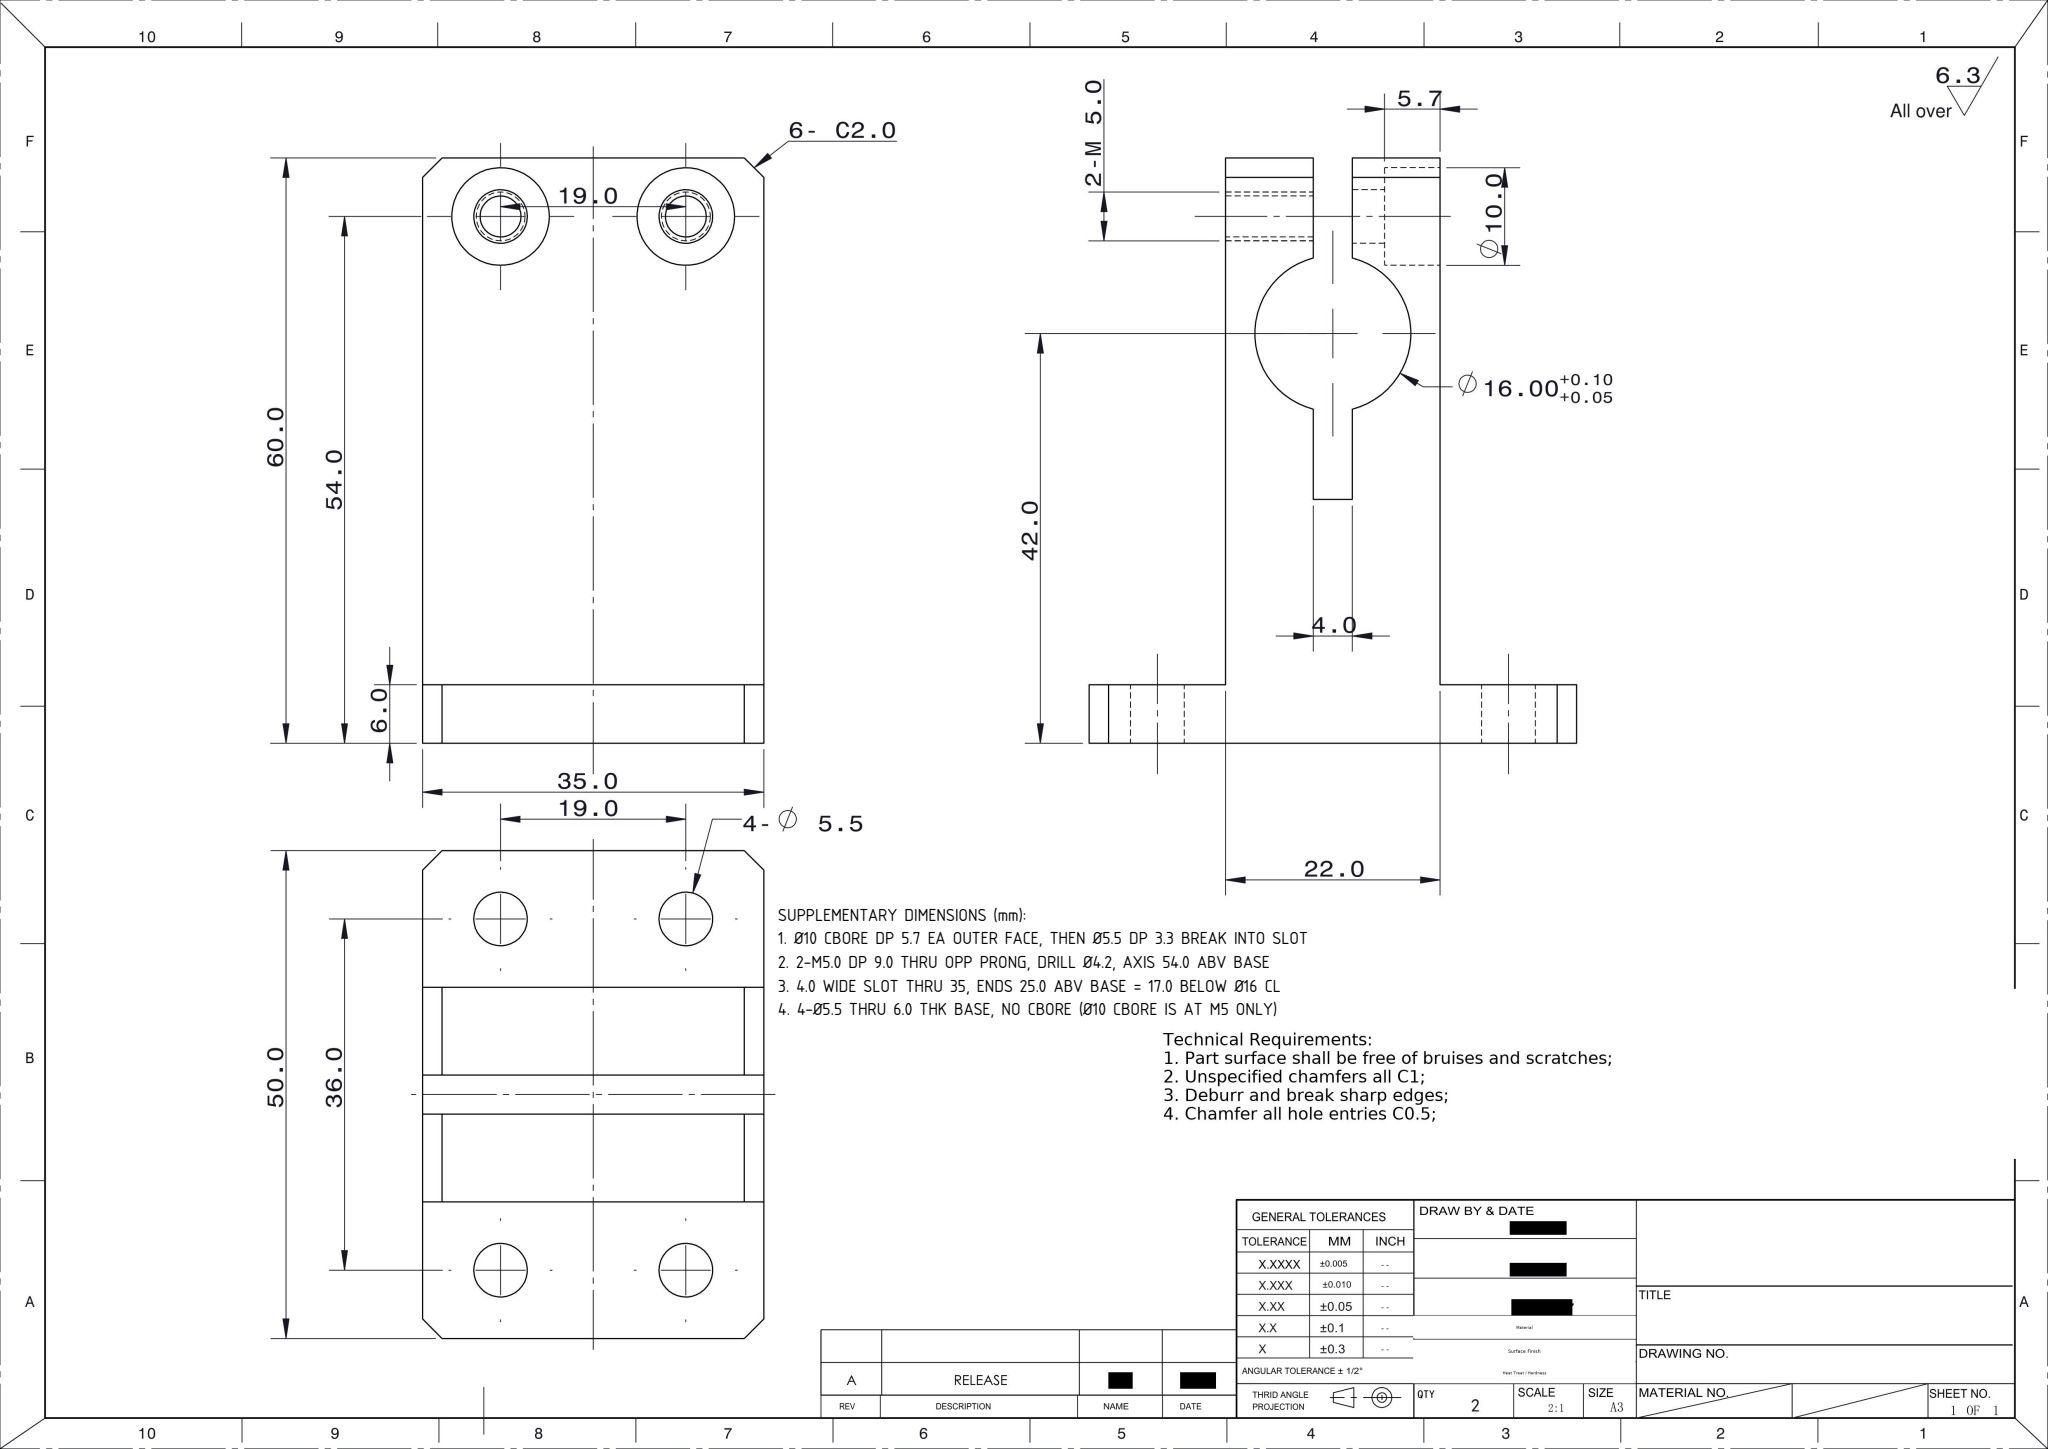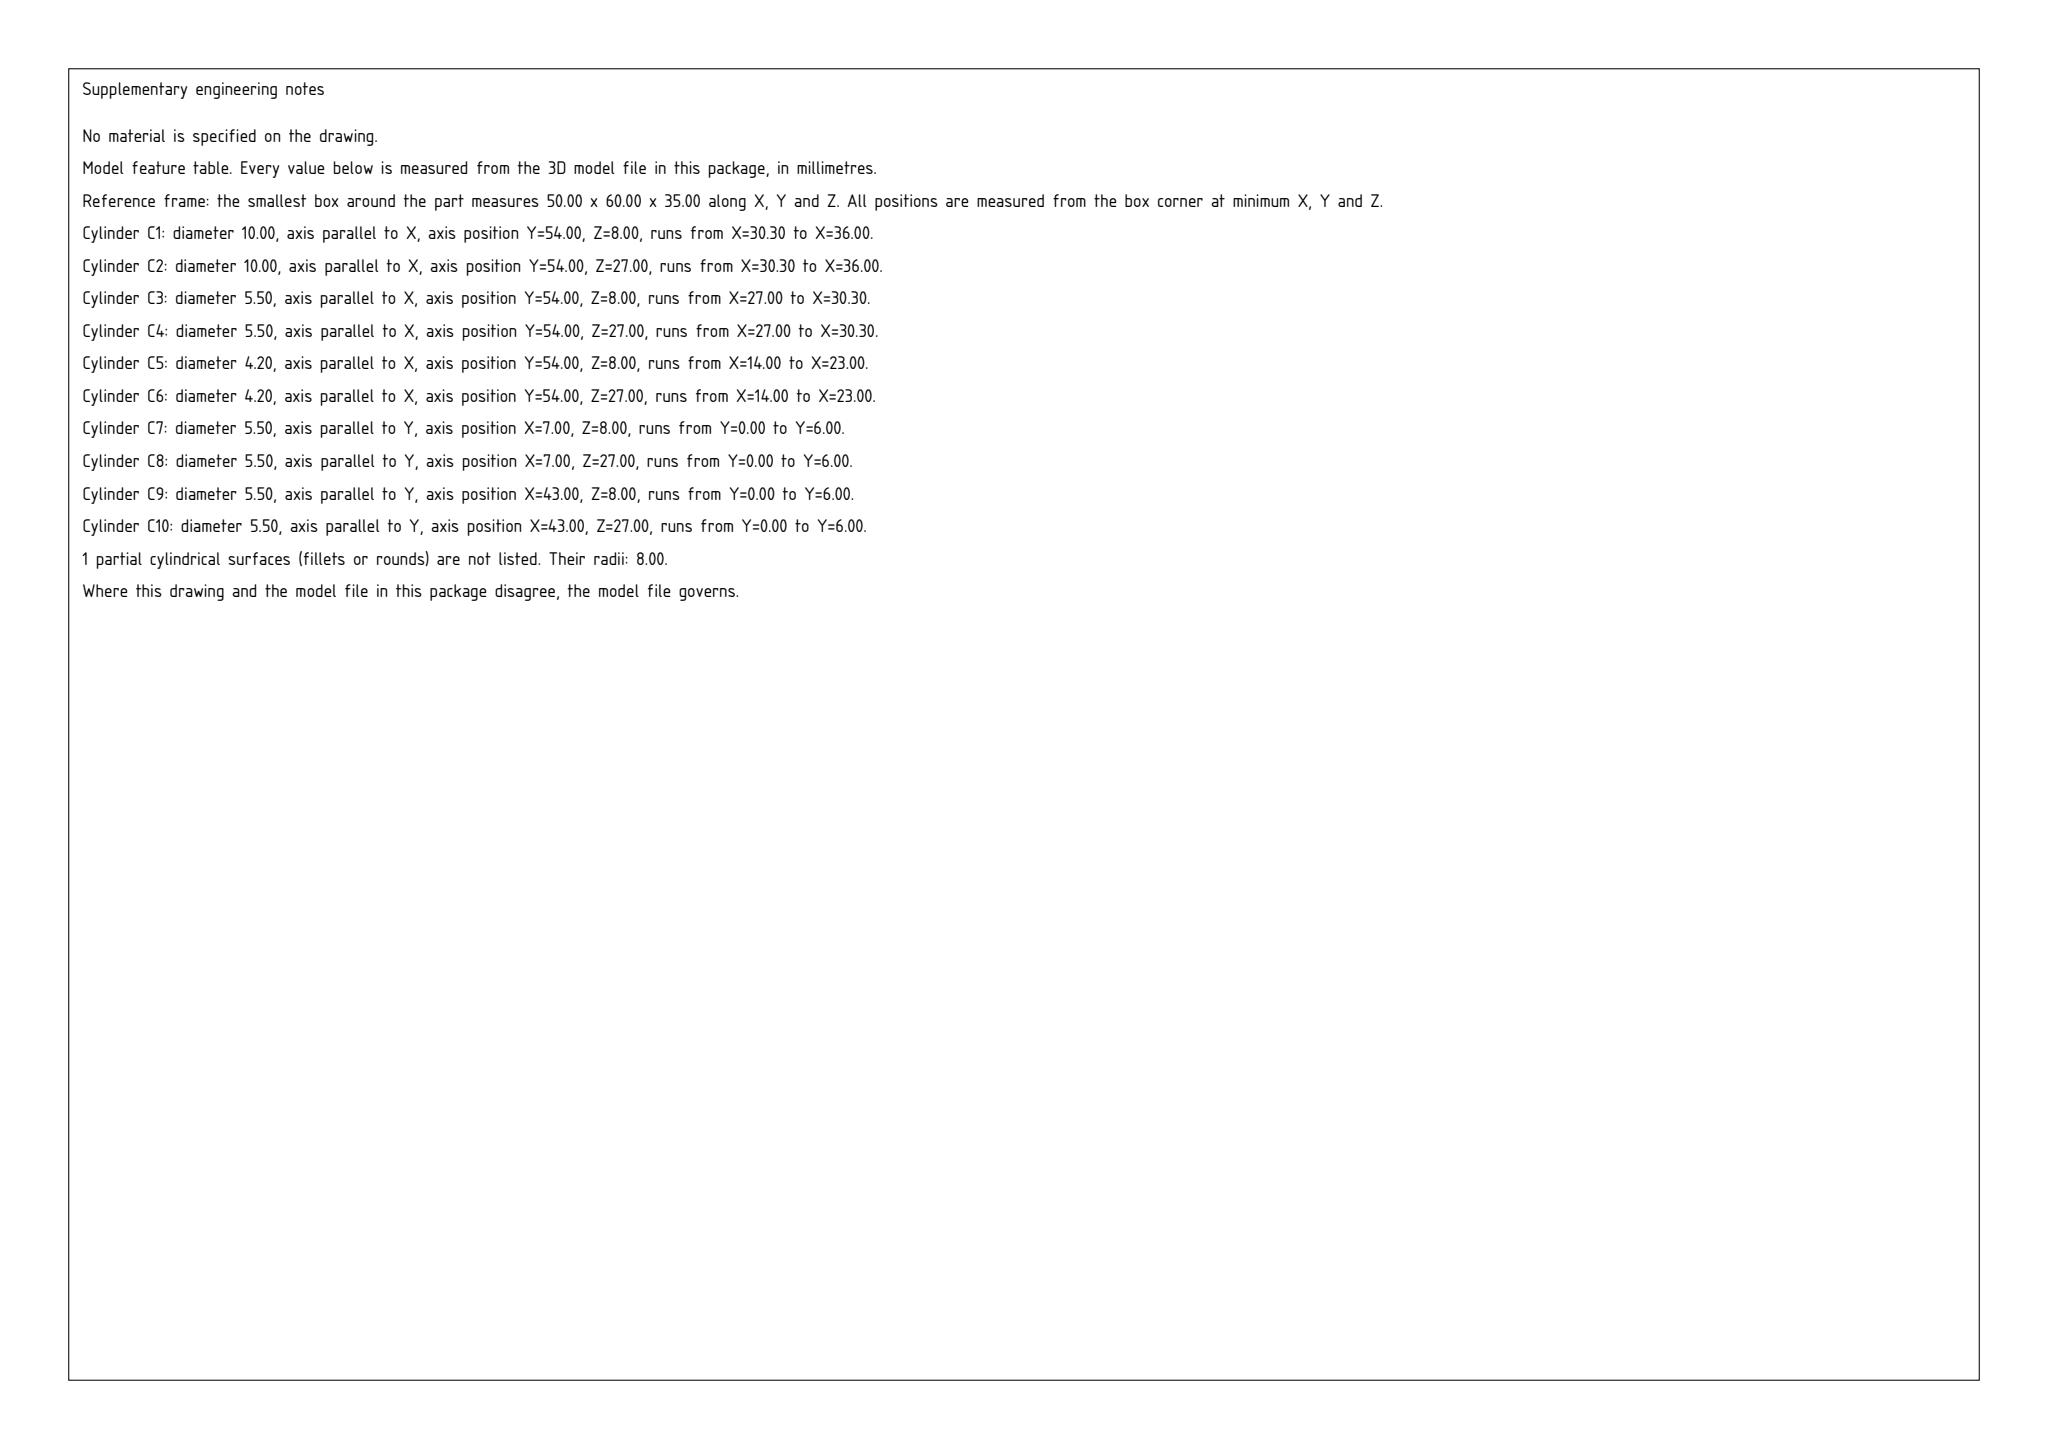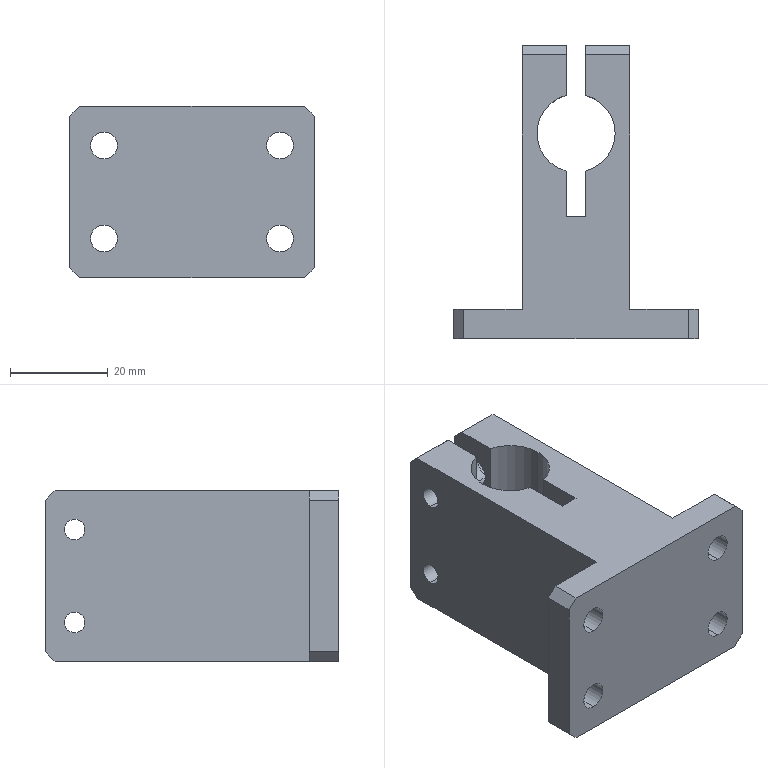Part | SolidWorks | mm | 1 solid | 49 faces | box 50 x 60 x 35 mm | volume 40368 mm3 | plane 26 | cylinder 23 | commonest cylinder face diameters 5.5 x12 4.2 x4 10 x4 16 x3
build123d program:
from build123d import *

# Parameters (mm, degrees)
SKETCH2_W                                         = 50
SKETCH2_H                                         = 60
BOSS_EXTRUDE1_DEPTH                               = 17.5
SKETCH3_W                                         = 14
SKETCH3_H                                         = 54
CUT_EXTRUDE1_DEPTH                                = 53.44
SKETCH5_R                                         = 8
CUT_EXTRUDE2_DEPTH                                = 53.44
SKETCH6_W                                         = 4
SKETCH6_H                                         = 70
CUT_EXTRUDE3_DEPTH                                = 53.44
HOLE_SIZE_ACCORDING_TO_HEXAGON_SOCKET_D           = 5.5
HOLE_SIZE_ACCORDING_TO_HEXAGON_SOCKET_DEPTH       = 9
HOLE_SIZE_ACCORDING_TO_HEXAGON_SOCKET_CBORE_D     = 10
HOLE_SIZE_ACCORDING_TO_HEXAGON_SOCKET_CBORE_DEPTH = 5.7
M5_TAPPED_HOLE1_D                                 = 4.2
M5_CLEARANCE_HOLE_1_D                             = 5.5
CHAMFER1_SIZE                                     = 2


with BuildPart() as part:
    # Sketch2 → Boss-Extrude1 (new, symmetric)
    with BuildSketch(Plane.XY):
        Rectangle(SKETCH2_W, SKETCH2_H)
    extrude(amount=BOSS_EXTRUDE1_DEPTH, both=True)

    # Sketch3 → Cut-Extrude1 (cut, through all)
    with BuildSketch(Plane.XY.offset(17.5)):
        with Locations((-18, 3)):
            Rectangle(SKETCH3_W, SKETCH3_H)
        with Locations((18, 3)):
            Rectangle(SKETCH3_W, SKETCH3_H)
    extrude(amount=-CUT_EXTRUDE1_DEPTH, mode=Mode.SUBTRACT)

    # Sketch5 → Cut-Extrude2 (cut, through all)
    with BuildSketch(Plane.XY.offset(17.5)):
        with Locations((0, 12)):
            Circle(SKETCH5_R)
    extrude(amount=-CUT_EXTRUDE2_DEPTH, mode=Mode.SUBTRACT)

    # Sketch6 → Cut-Extrude3 (cut, through all)
    with BuildSketch(Plane.XY.offset(17.5)):
        with Locations((0, 30)):
            Rectangle(SKETCH6_W, SKETCH6_H)
    extrude(amount=-CUT_EXTRUDE3_DEPTH, mode=Mode.SUBTRACT)

    # Hole Size _ according to_ Hexagon Socket
    with Locations(Plane(origin=(11, 0, 0), x_dir=(0, 0, -1), z_dir=(1, 0, 0))):
        with Locations((-9.5, 24), (9.5, 24)):
            CounterBoreHole(HOLE_SIZE_ACCORDING_TO_HEXAGON_SOCKET_D / 2, HOLE_SIZE_ACCORDING_TO_HEXAGON_SOCKET_CBORE_D / 2, HOLE_SIZE_ACCORDING_TO_HEXAGON_SOCKET_CBORE_DEPTH, depth=HOLE_SIZE_ACCORDING_TO_HEXAGON_SOCKET_DEPTH)

    # M5 Tapped Hole1 (through all)
    with Locations(Plane(origin=(-2, 0, 0), x_dir=(0, 0, -1), z_dir=(1, 0, 0))):
        with Locations((-9.5, 24), (9.5, 24)):
            Hole(M5_TAPPED_HOLE1_D / 2)

    # M5 Clearance Hole 1 (through all)
    with Locations(Plane(origin=(0, -24, 0), x_dir=(1, 0, 0), z_dir=(0, 1, 0))):
        with Locations((-18, 9.5), (-18, -9.5), (18, 9.5), (18, -9.5)):
            Hole(M5_CLEARANCE_HOLE_1_D / 2)

    # Chamfer1
    chamfer1_edges = [part.edges().sort_by_distance(p)[0] for p in [
        (25, -27, 17.5),
        (-25, -27, -17.5),
        (-25, -27, 17.5),
        (6.5, 30, -17.5),
        (6.5, 30, 17.5),
        (25, -27, -17.5),
        (-6.5, 30, -17.5),
        (-6.5, 30, 17.5),
    ]]
    chamfer(chamfer1_edges, length=CHAMFER1_SIZE)


solid = part.part